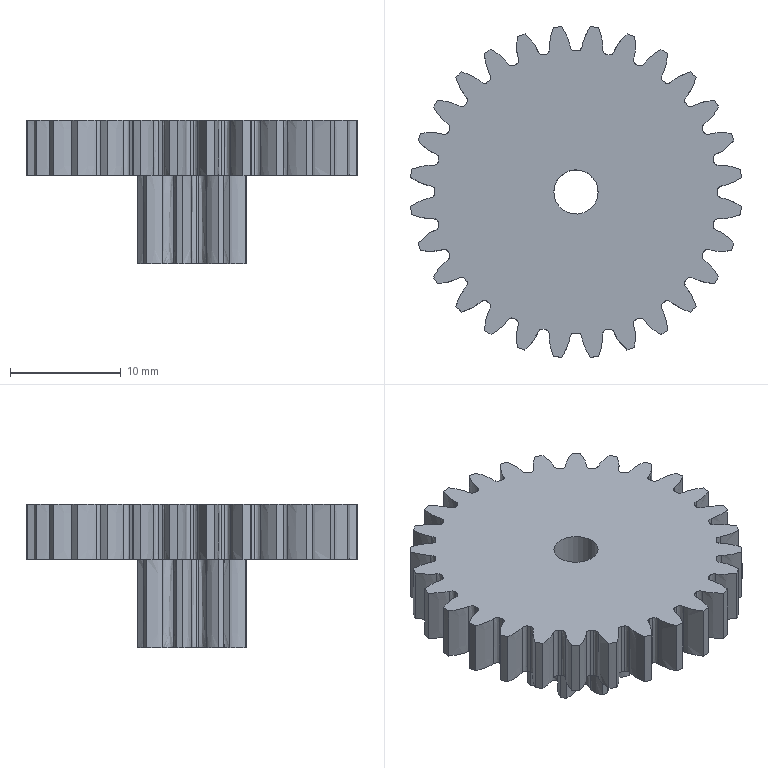Component | NX | GEAR_2 | 1 solid | 220 faces | volume 3260 mm3 | other 180 | cylinder 37 | plane 3 | commonest cylinder face diameters 25.5 x28 5.5 x8 4 x1